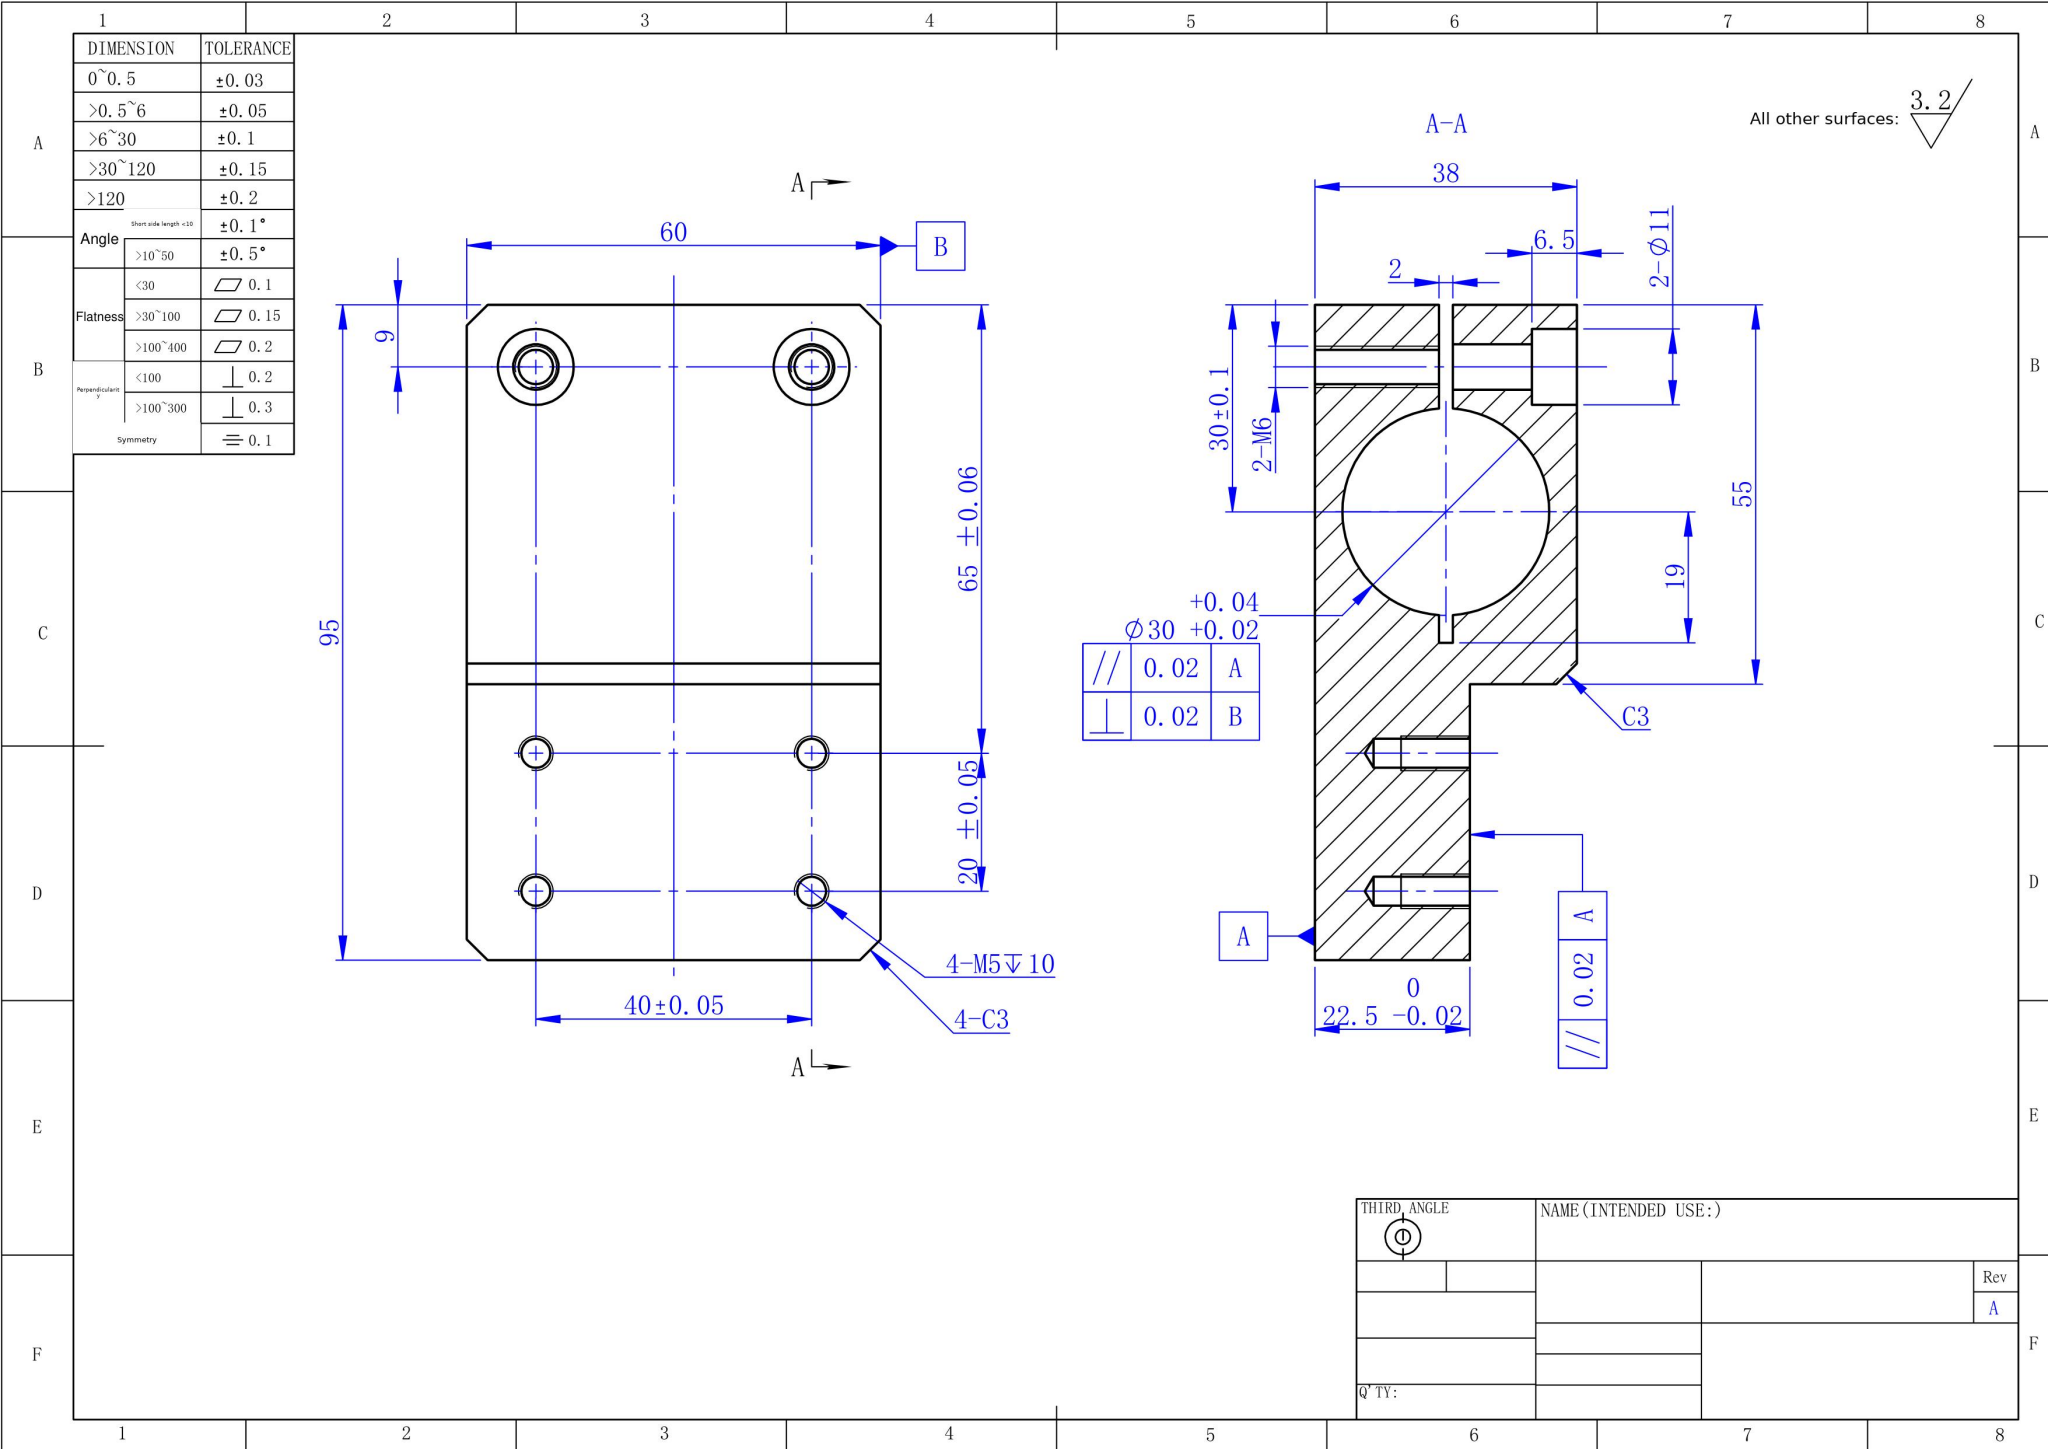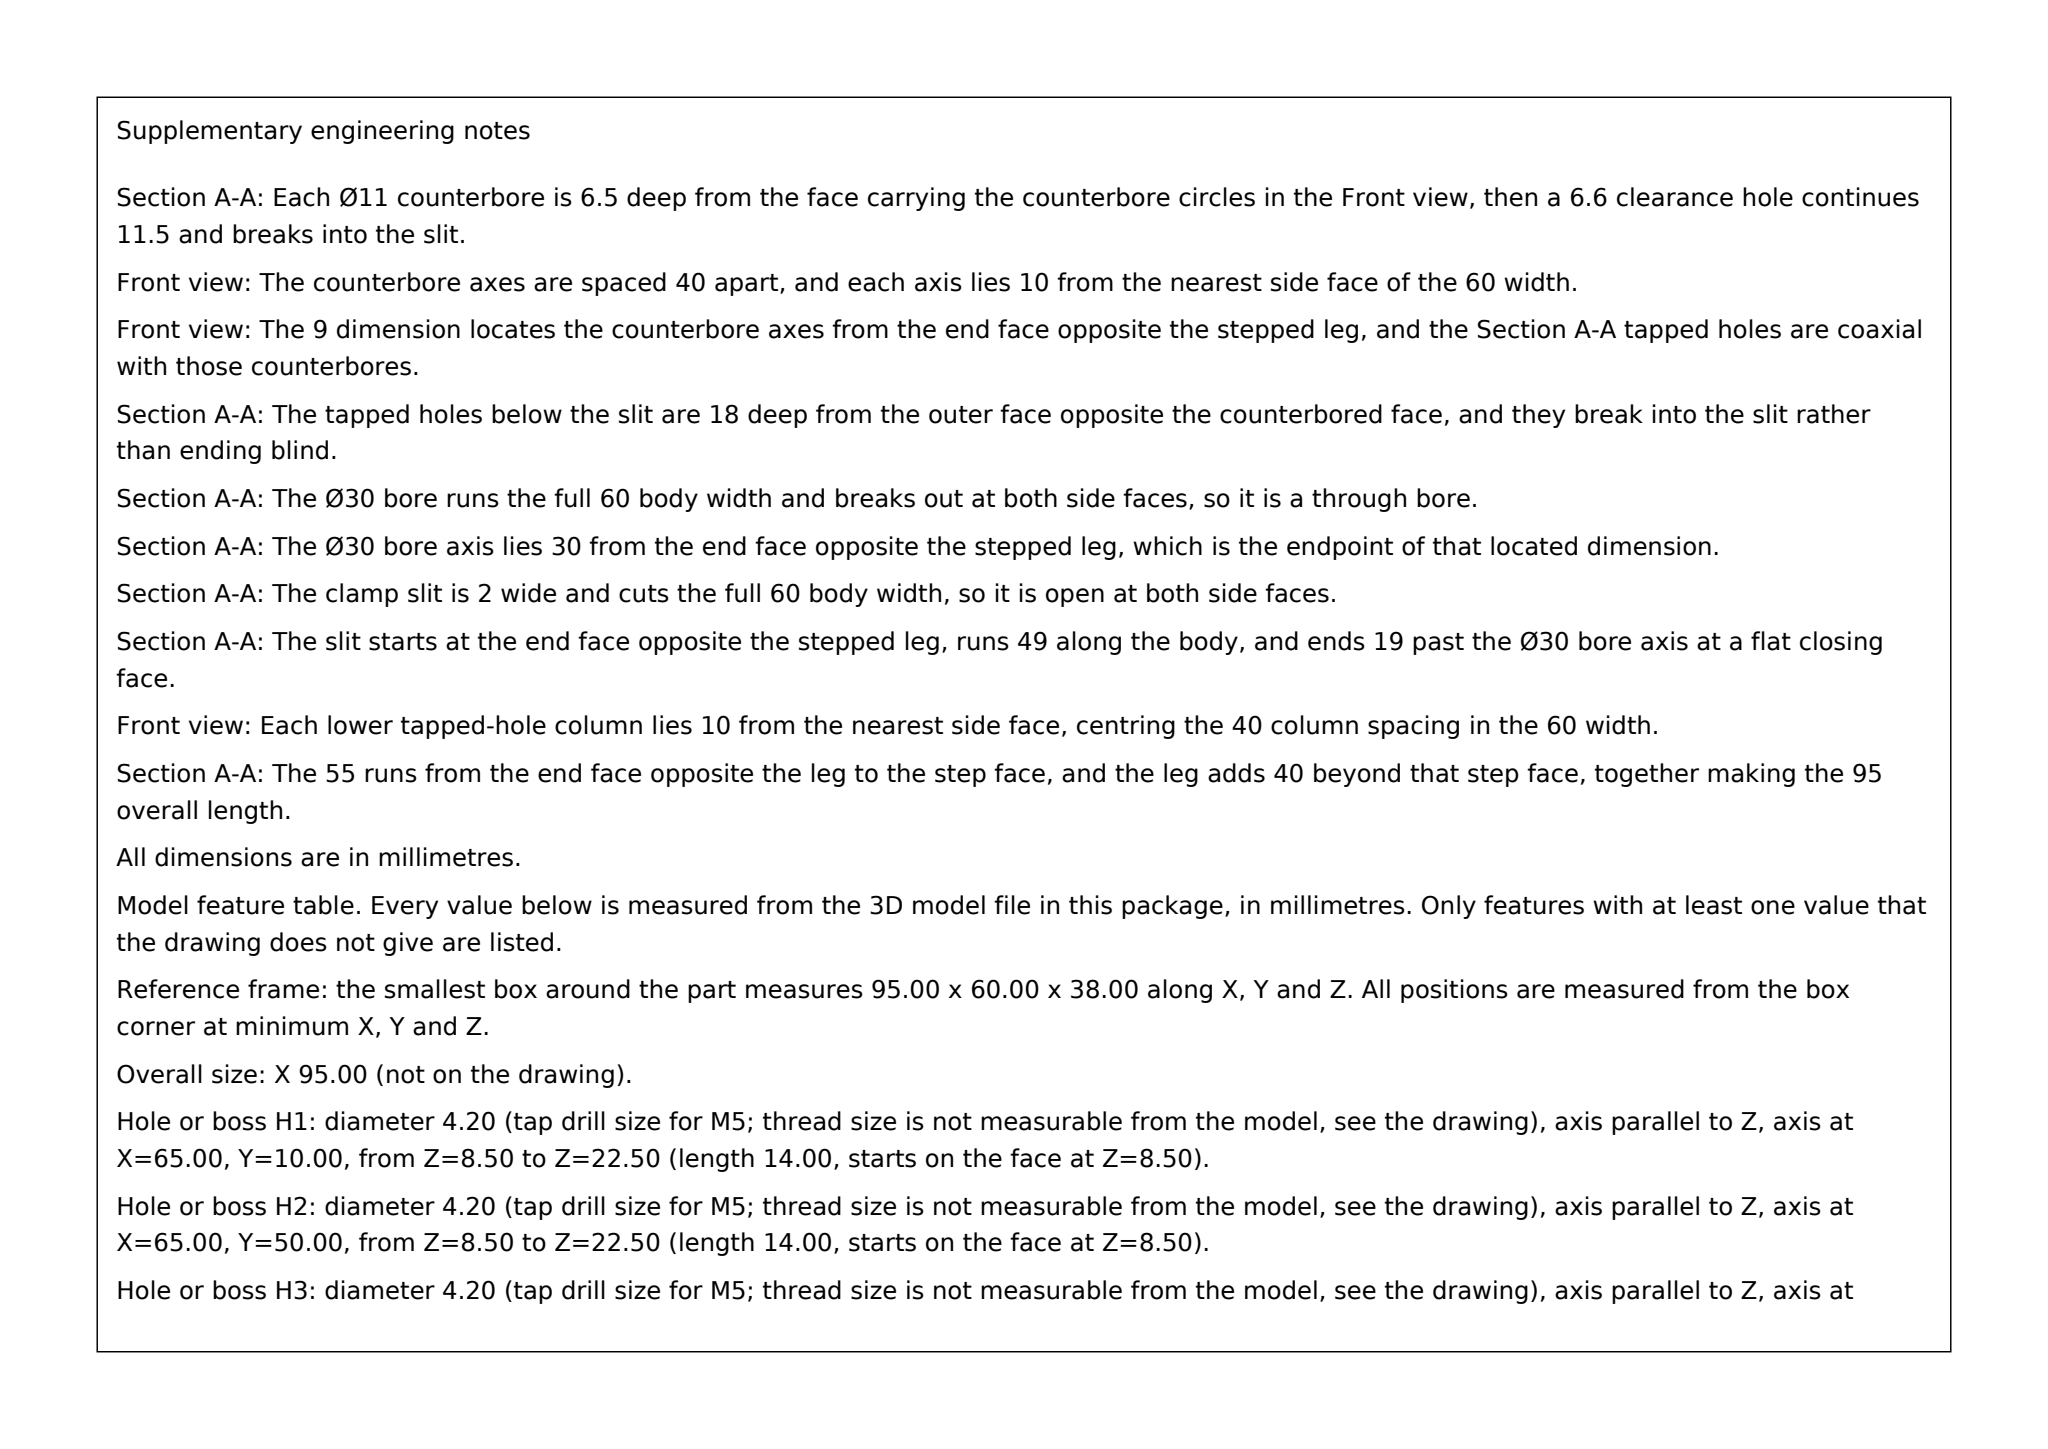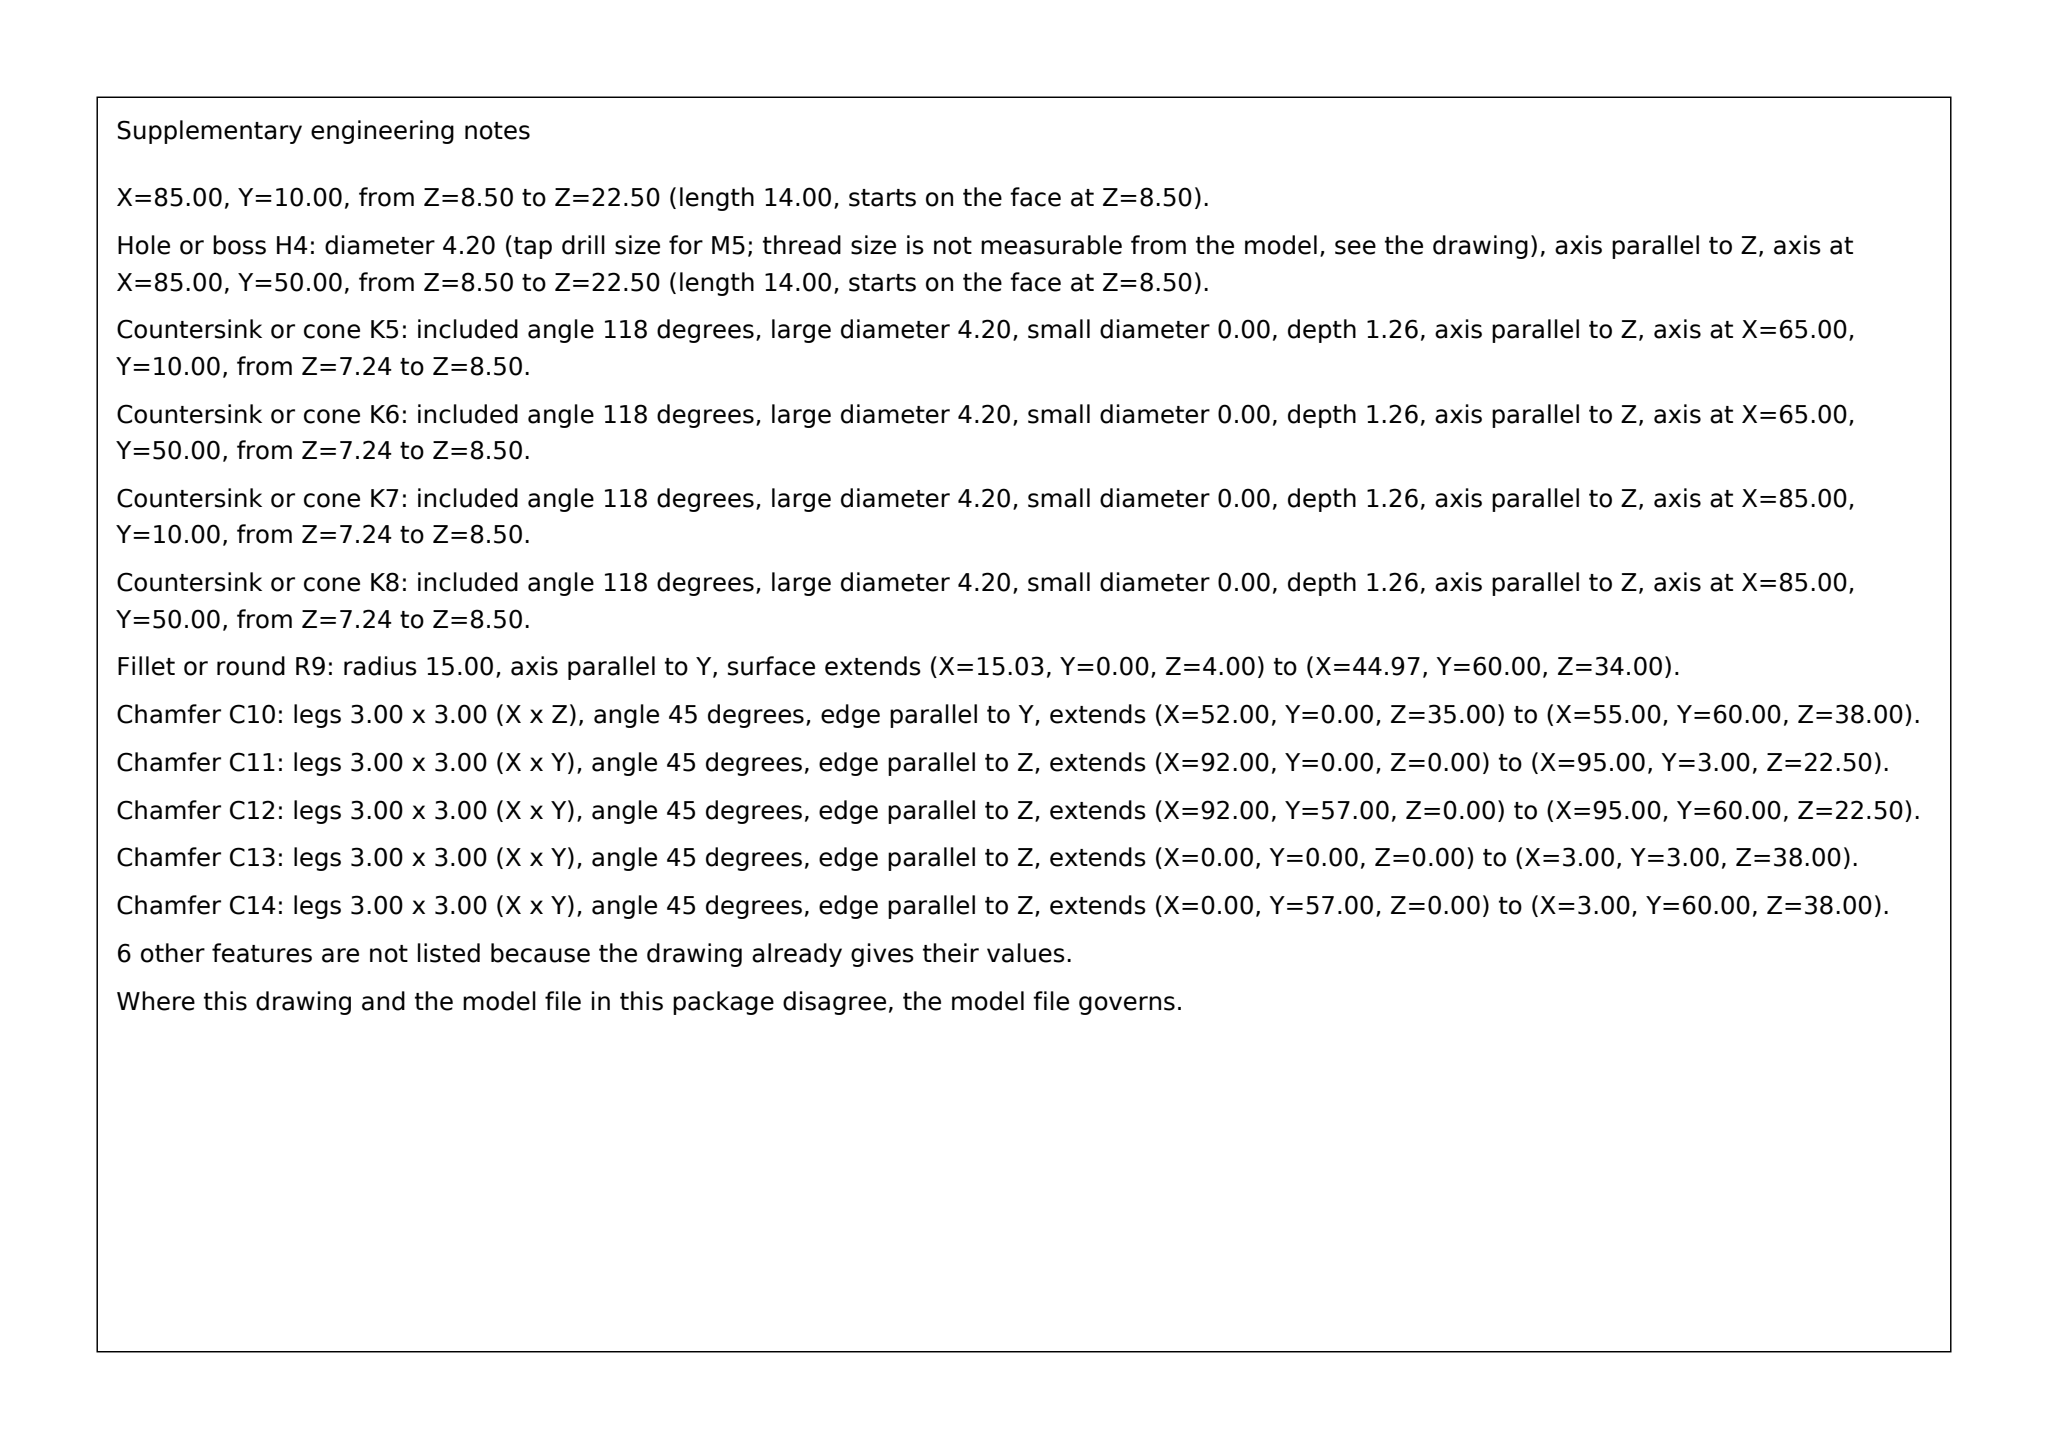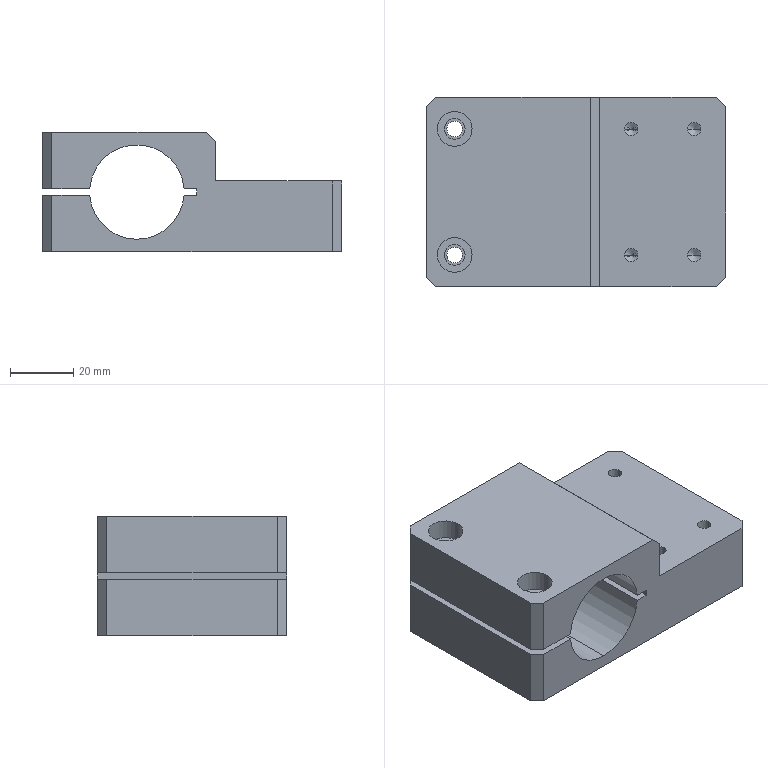Part | SolidWorks | mm | 1 solid | 54 faces | box 95 x 60 x 38 mm | volume 130381 mm3 | cylinder 23 | plane 23 | cone 8 | commonest cylinder face diameters 4.2 x8 5 x4 11 x4 6.6 x4 30 x3
Drawing notes:
Ø30 BORE THRU 60 WIDE; AXIS 19 FROM DATUM A FACE = MID OF 38 THK | from the solid: Ø30 cylinder axis y, length 60, pos x=30, z=19; bbox z=38, datum A face z=0
2 WIDE CLAMP SLIT 18 FROM DATUM A FACE, CL ON Ø30 BORE AXIS | from the solid: z-normal planes at 18 and 20 (2 wide); midplane z=19 = Ø30 bore axis z=19
2-M6 TAP DRILL Ø5 DP 18 FROM DATUM A FACE THRU TO SLIT; 40 APART, 9 FROM TOP | from the solid: Ø5 z-holes at x=9, y=10 & 50, length 18 from z=0 to slit face z=18; spacing 50-10=40
2X Ø6.6 DP 11.5 FROM SLIT FACE, 40 APART, 9 FROM TOP | from the solid: Ø6.6 z-holes at x=9, y=10 & 50, length 11.5 from z=20 to z=31.5
2-Ø11 CBORE DP 6.5 FROM FACE OPP DATUM A, 40 APART | from the solid: Ø11 z-holes at x=9, y=10 & 50, length 6.5 from z=38 face to z=31.5
2 WIDE CLAMP SLIT: EXTENDS 49 FROM TOP FACE (4 BEYOND Ø30 BORE) | from the solid: axis_plane x=49 (slit relief bottom); Ø30 bore axis at x=30, bore bottom x=45; slit width 2 from top face x=0
build123d program:
from build123d import *

# Parameters (mm, degrees)
BOSS_EXTRUDE1_DEPTH                             = 60
M6_HEX_SOCKET_HEAD_CAP_SCREW_CBORE1_D           = 6.6
M6_HEX_SOCKET_HEAD_CAP_SCREW_CBORE1_DEPTH       = 18
M6_HEX_SOCKET_HEAD_CAP_SCREW_CBORE1_CBORE_D     = 11
M6_HEX_SOCKET_HEAD_CAP_SCREW_CBORE1_CBORE_DEPTH = 6.5
M6_TAPPED_HOLE1_D                               = 5
M5_TAPPED_HOLE1_D                               = 4.2
M5_TAPPED_HOLE1_DEPTH                           = 14
M5_TAPPED_HOLE1_TIP                             = 1.262
CHAMFER1_SIZE                                   = 3


with BuildPart() as part:
    # Sketch1 → Boss-Extrude1 (new body)
    with BuildSketch(Plane(origin=(0, 0, 0), x_dir=(1, 0, 0), z_dir=(0, 1, 0))):
        with BuildLine():
            Line((25, -3.5), (65, -3.5))
            Line((65, -3.5), (65, 19))
            Line((65, 19), (-30, 19))
            Line((-30, 19), (-30, 1))
            Line((-30, 1), (-14.967, 1))
            ThreePointArc((-14.967, 1), (0, 15), (14.967, 1))
            Line((14.967, 1), (19, 1))
            Line((19, 1), (19, -1))
            Line((19, -1), (14.967, -1))
            ThreePointArc((14.967, -1), (0, -15), (-14.967, -1))
            Line((-14.967, -1), (-30, -1))
            Line((-30, -1), (-30, -19))
            Line((-30, -19), (25, -19))
            Line((25, -19), (25, -3.5))
        make_face()
    extrude(amount=BOSS_EXTRUDE1_DEPTH)

    # M6 Hex Socket Head Cap Screw CBORE1
    with Locations(Plane.XY.offset(19)):
        with Locations((-21, 50), (-21, 10)):
            CounterBoreHole(M6_HEX_SOCKET_HEAD_CAP_SCREW_CBORE1_D / 2, M6_HEX_SOCKET_HEAD_CAP_SCREW_CBORE1_CBORE_D / 2, M6_HEX_SOCKET_HEAD_CAP_SCREW_CBORE1_CBORE_DEPTH, depth=M6_HEX_SOCKET_HEAD_CAP_SCREW_CBORE1_DEPTH)

    # M6 Tapped Hole1 (through all)
    with Locations(Plane.XY.offset(-1)):
        with Locations((-21, 50), (-21, 10)):
            Hole(M6_TAPPED_HOLE1_D / 2)

    # M5 Tapped Hole1
    with Locations(Plane.XY.offset(3.5)):
        with Locations((35, 50), (55, 10), (35, 10), (55, 50)):
            Hole(M5_TAPPED_HOLE1_D / 2, depth=M5_TAPPED_HOLE1_DEPTH)
            with Locations((0, 0, -(M5_TAPPED_HOLE1_DEPTH + M5_TAPPED_HOLE1_TIP / 2))):  # 118° drill point
                Cone(0, M5_TAPPED_HOLE1_D / 2, M5_TAPPED_HOLE1_TIP, mode=Mode.SUBTRACT)

    # Chamfer1
    chamfer1_edges = [part.edges().sort_by_distance(p)[0] for p in [
        (-30, 0, -10),
        (65, 0, -7.75),
        (-30, 60, 10),
        (-30, 0, 10),
        (25, 30, 19),
        (65, 60, -7.75),
        (-30, 60, -10),
    ]]
    chamfer(chamfer1_edges, length=CHAMFER1_SIZE)


solid = part.part